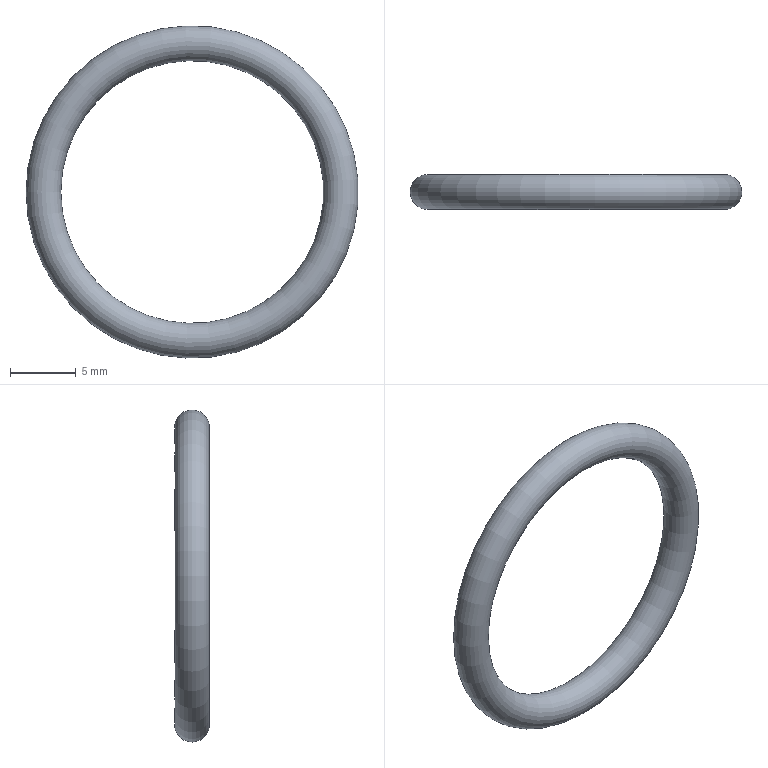Component | NX | O_RING_20 | 1 solid | 1 faces | box 25.3 x 2.65 x 25.3 mm | volume 392 mm3 | torus 1
STEP:
#1=CARTESIAN_POINT('',(0.,0.,0.));
#2=DIRECTION('',(0.,0.,1.));
#3=DIRECTION('',(1.,0.,0.));
#4=AXIS2_PLACEMENT_3D('',#1,#2,#3);
#5=CARTESIAN_POINT('',(-12.65,-7.425,43.));
#6=VERTEX_POINT('',#5);
#7=CARTESIAN_POINT('',(-11.325,-7.425,43.));
#8=DIRECTION('',(0.,0.,-1.));
#9=DIRECTION('',(-1.,0.,0.));
#10=AXIS2_PLACEMENT_3D('',#7,#8,#9);
#11=CIRCLE('',#10,1.325);
#12=CARTESIAN_POINT('',(0.,-7.425,43.));
#13=DIRECTION('',(0.,1.,0.));
#14=DIRECTION('',(-1.,0.,0.));
#15=AXIS2_PLACEMENT_3D('',#12,#13,#14);
#16=TOROIDAL_SURFACE('',#15,11.325,1.325);
#17=CARTESIAN_POINT('',(0.,0.));
#18=DIRECTION('',(0.,1.));
#19=VECTOR('',#18,1.);
#20=LINE('',#17,#19);
#21=(GEOMETRIC_REPRESENTATION_CONTEXT(2)PARAMETRIC_REPRESENTATION_CONTEXT()REPRESENTATION_CONTEXT('',''));
#22=DEFINITIONAL_REPRESENTATION('',(#20),#21);
#23=PCURVE('',#16,#22);
#24=CARTESIAN_POINT('',(6.283,0.));
#25=DIRECTION('',(0.,1.));
#26=VECTOR('',#25,1.);
#27=LINE('',#24,#26);
#28=(GEOMETRIC_REPRESENTATION_CONTEXT(2)PARAMETRIC_REPRESENTATION_CONTEXT()REPRESENTATION_CONTEXT('',''));
#29=DEFINITIONAL_REPRESENTATION('',(#27),#28);
#30=PCURVE('',#16,#29);
#31=SEAM_CURVE('',#11,(#23,#30),.PCURVE_S1.);
#32=EDGE_CURVE('',#6,#6,#31,.T.);
#33=ORIENTED_EDGE('',*,*,#32,.F.);
#34=CARTESIAN_POINT('',(0.,-7.425,43.));
#35=DIRECTION('',(0.,1.,0.));
#36=DIRECTION('',(-1.,0.,0.));
#37=AXIS2_PLACEMENT_3D('',#34,#35,#36);
#38=CIRCLE('',#37,12.65);
#39=CARTESIAN_POINT('',(0.,0.));
#40=DIRECTION('',(1.,0.));
#41=VECTOR('',#40,1.);
#42=LINE('',#39,#41);
#43=(GEOMETRIC_REPRESENTATION_CONTEXT(2)PARAMETRIC_REPRESENTATION_CONTEXT()REPRESENTATION_CONTEXT('',''));
#44=DEFINITIONAL_REPRESENTATION('',(#42),#43);
#45=PCURVE('',#16,#44);
#46=CARTESIAN_POINT('',(0.,6.283));
#47=DIRECTION('',(1.,0.));
#48=VECTOR('',#47,1.);
#49=LINE('',#46,#48);
#50=(GEOMETRIC_REPRESENTATION_CONTEXT(2)PARAMETRIC_REPRESENTATION_CONTEXT()REPRESENTATION_CONTEXT('',''));
#51=DEFINITIONAL_REPRESENTATION('',(#49),#50);
#52=PCURVE('',#16,#51);
#53=SEAM_CURVE('',#38,(#45,#52),.PCURVE_S1.);
#54=EDGE_CURVE('',#6,#6,#53,.T.);
#55=ORIENTED_EDGE('',*,*,#54,.T.);
#56=ORIENTED_EDGE('',*,*,#32,.T.);
#57=ORIENTED_EDGE('',*,*,#54,.F.);
#58=EDGE_LOOP('',(#33,#55,#56,#57));
#59=FACE_BOUND('',#58,.T.);
#60=ADVANCED_FACE('',(#59),#16,.T.);
#61=CLOSED_SHELL('',(#60));
#62=MANIFOLD_SOLID_BREP('',#61);
#63=(LENGTH_UNIT()NAMED_UNIT(*)SI_UNIT(.MILLI.,.METRE.));
#64=UNCERTAINTY_MEASURE_WITH_UNIT(LENGTH_MEASURE(0.0000001),#63,'','');
#65=(NAMED_UNIT(*)PLANE_ANGLE_UNIT()SI_UNIT($,.RADIAN.));
#66=(NAMED_UNIT(*)SI_UNIT($,.STERADIAN.)SOLID_ANGLE_UNIT());
#67=(GEOMETRIC_REPRESENTATION_CONTEXT(3)GLOBAL_UNCERTAINTY_ASSIGNED_CONTEXT((#64))GLOBAL_UNIT_ASSIGNED_CONTEXT((#63,#65,#66))REPRESENTATION_CONTEXT('',''));
#68=ADVANCED_BREP_SHAPE_REPRESENTATION('',(#4,#62),#67);